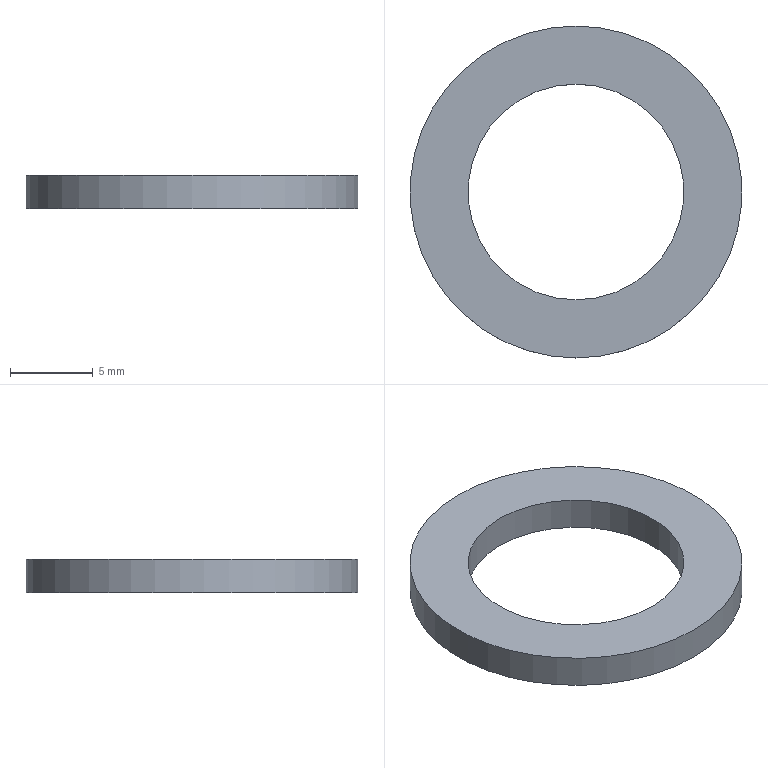Component | NX | GB-T848-2002_M12 | 1 solid | 4 faces | box 20 x 20 x 2 mm | volume 363 mm3 | cylinder 2 | plane 2 | commonest cylinder face diameters 20 x1 13 x1
STEP:
#1=CARTESIAN_POINT('',(0.,0.,0.));
#2=DIRECTION('',(0.,0.,1.));
#3=DIRECTION('',(1.,0.,0.));
#4=AXIS2_PLACEMENT_3D('',#1,#2,#3);
#5=CARTESIAN_POINT('',(0.,10.,-15.));
#6=VERTEX_POINT('',#5);
#7=CARTESIAN_POINT('',(0.,0.,-15.));
#8=DIRECTION('',(0.,0.,-1.));
#9=DIRECTION('',(0.,1.,0.));
#10=AXIS2_PLACEMENT_3D('',#7,#8,#9);
#11=CIRCLE('',#10,10.);
#12=CARTESIAN_POINT('',(0.,0.,-15.));
#13=DIRECTION('',(0.,0.,1.));
#14=DIRECTION('',(0.,-1.,0.));
#15=AXIS2_PLACEMENT_3D('',#12,#13,#14);
#16=CYLINDRICAL_SURFACE('',#15,10.);
#17=CARTESIAN_POINT('',(9.425,0.));
#18=DIRECTION('',(-1.,0.));
#19=VECTOR('',#18,1.);
#20=LINE('',#17,#19);
#21=(GEOMETRIC_REPRESENTATION_CONTEXT(2)PARAMETRIC_REPRESENTATION_CONTEXT()REPRESENTATION_CONTEXT('',''));
#22=DEFINITIONAL_REPRESENTATION('',(#20),#21);
#23=PCURVE('',#16,#22);
#24=CARTESIAN_POINT('',(0.,0.,-15.));
#25=DIRECTION('',(0.,0.,-1.));
#26=DIRECTION('',(0.,1.,0.));
#27=AXIS2_PLACEMENT_3D('',#24,#25,#26);
#28=PLANE('',#27);
#29=CARTESIAN_POINT('',(0.,0.));
#30=DIRECTION('',(1.,0.));
#31=AXIS2_PLACEMENT_2D('',#29,#30);
#32=CIRCLE('',#31,10.);
#33=(GEOMETRIC_REPRESENTATION_CONTEXT(2)PARAMETRIC_REPRESENTATION_CONTEXT()REPRESENTATION_CONTEXT('',''));
#34=DEFINITIONAL_REPRESENTATION('',(#32),#33);
#35=PCURVE('',#28,#34);
#36=SURFACE_CURVE('',#11,(#23,#35),.PCURVE_S1.);
#37=EDGE_CURVE('',#6,#6,#36,.T.);
#38=ORIENTED_EDGE('',*,*,#37,.F.);
#39=CARTESIAN_POINT('',(0.,10.,-13.));
#40=VERTEX_POINT('',#39);
#41=CARTESIAN_POINT('',(0.,10.,-15.));
#42=CARTESIAN_POINT('',(0.,10.,-13.));
#43=B_SPLINE_CURVE_WITH_KNOTS('',1,(#41,#42),.UNSPECIFIED.,.F.,.F.,(2,2),(0.,2.),.PIECEWISE_BEZIER_KNOTS.);
#44=CARTESIAN_POINT('',(9.425,0.));
#45=DIRECTION('',(0.,1.));
#46=VECTOR('',#45,1.);
#47=LINE('',#44,#46);
#48=(GEOMETRIC_REPRESENTATION_CONTEXT(2)PARAMETRIC_REPRESENTATION_CONTEXT()REPRESENTATION_CONTEXT('',''));
#49=DEFINITIONAL_REPRESENTATION('',(#47),#48);
#50=PCURVE('',#16,#49);
#51=CARTESIAN_POINT('',(3.142,0.));
#52=DIRECTION('',(0.,1.));
#53=VECTOR('',#52,1.);
#54=LINE('',#51,#53);
#55=(GEOMETRIC_REPRESENTATION_CONTEXT(2)PARAMETRIC_REPRESENTATION_CONTEXT()REPRESENTATION_CONTEXT('',''));
#56=DEFINITIONAL_REPRESENTATION('',(#54),#55);
#57=PCURVE('',#16,#56);
#58=SEAM_CURVE('',#43,(#50,#57),.PCURVE_S1.);
#59=EDGE_CURVE('',#6,#40,#58,.T.);
#60=ORIENTED_EDGE('',*,*,#59,.T.);
#61=CARTESIAN_POINT('',(0.,0.,-13.));
#62=DIRECTION('',(0.,0.,-1.));
#63=DIRECTION('',(0.,1.,0.));
#64=AXIS2_PLACEMENT_3D('',#61,#62,#63);
#65=CIRCLE('',#64,10.);
#66=CARTESIAN_POINT('',(9.425,2.));
#67=DIRECTION('',(-1.,0.));
#68=VECTOR('',#67,1.);
#69=LINE('',#66,#68);
#70=(GEOMETRIC_REPRESENTATION_CONTEXT(2)PARAMETRIC_REPRESENTATION_CONTEXT()REPRESENTATION_CONTEXT('',''));
#71=DEFINITIONAL_REPRESENTATION('',(#69),#70);
#72=PCURVE('',#16,#71);
#73=CARTESIAN_POINT('',(0.,0.,-13.));
#74=DIRECTION('',(0.,0.,-1.));
#75=DIRECTION('',(0.,1.,0.));
#76=AXIS2_PLACEMENT_3D('',#73,#74,#75);
#77=PLANE('',#76);
#78=CARTESIAN_POINT('',(0.,0.));
#79=DIRECTION('',(1.,0.));
#80=AXIS2_PLACEMENT_2D('',#78,#79);
#81=CIRCLE('',#80,10.);
#82=(GEOMETRIC_REPRESENTATION_CONTEXT(2)PARAMETRIC_REPRESENTATION_CONTEXT()REPRESENTATION_CONTEXT('',''));
#83=DEFINITIONAL_REPRESENTATION('',(#81),#82);
#84=PCURVE('',#77,#83);
#85=SURFACE_CURVE('',#65,(#72,#84),.PCURVE_S1.);
#86=EDGE_CURVE('',#40,#40,#85,.T.);
#87=ORIENTED_EDGE('',*,*,#86,.T.);
#88=ORIENTED_EDGE('',*,*,#59,.F.);
#89=EDGE_LOOP('',(#38,#60,#87,#88));
#90=FACE_BOUND('',#89,.T.);
#91=ADVANCED_FACE('',(#90),#16,.T.);
#92=CARTESIAN_POINT('',(0.,6.5,-15.));
#93=VERTEX_POINT('',#92);
#94=CARTESIAN_POINT('',(0.,0.,-15.));
#95=DIRECTION('',(0.,0.,-1.));
#96=DIRECTION('',(0.,1.,0.));
#97=AXIS2_PLACEMENT_3D('',#94,#95,#96);
#98=CIRCLE('',#97,6.5);
#99=CARTESIAN_POINT('',(0.,0.,-15.));
#100=DIRECTION('',(0.,0.,1.));
#101=DIRECTION('',(0.,-1.,0.));
#102=AXIS2_PLACEMENT_3D('',#99,#100,#101);
#103=CYLINDRICAL_SURFACE('',#102,6.5);
#104=CARTESIAN_POINT('',(9.425,0.));
#105=DIRECTION('',(-1.,0.));
#106=VECTOR('',#105,1.);
#107=LINE('',#104,#106);
#108=(GEOMETRIC_REPRESENTATION_CONTEXT(2)PARAMETRIC_REPRESENTATION_CONTEXT()REPRESENTATION_CONTEXT('',''));
#109=DEFINITIONAL_REPRESENTATION('',(#107),#108);
#110=PCURVE('',#103,#109);
#111=CARTESIAN_POINT('',(0.,0.));
#112=DIRECTION('',(1.,0.));
#113=AXIS2_PLACEMENT_2D('',#111,#112);
#114=CIRCLE('',#113,6.5);
#115=(GEOMETRIC_REPRESENTATION_CONTEXT(2)PARAMETRIC_REPRESENTATION_CONTEXT()REPRESENTATION_CONTEXT('',''));
#116=DEFINITIONAL_REPRESENTATION('',(#114),#115);
#117=PCURVE('',#28,#116);
#118=SURFACE_CURVE('',#98,(#110,#117),.PCURVE_S1.);
#119=EDGE_CURVE('',#93,#93,#118,.T.);
#120=ORIENTED_EDGE('',*,*,#119,.F.);
#121=CARTESIAN_POINT('',(0.,6.5,-13.));
#122=VERTEX_POINT('',#121);
#123=CARTESIAN_POINT('',(0.,6.5,-15.));
#124=CARTESIAN_POINT('',(0.,6.5,-13.));
#125=B_SPLINE_CURVE_WITH_KNOTS('',1,(#123,#124),.UNSPECIFIED.,.F.,.F.,(2,2),(0.,2.),.PIECEWISE_BEZIER_KNOTS.);
#126=CARTESIAN_POINT('',(9.425,0.));
#127=DIRECTION('',(0.,1.));
#128=VECTOR('',#127,1.);
#129=LINE('',#126,#128);
#130=(GEOMETRIC_REPRESENTATION_CONTEXT(2)PARAMETRIC_REPRESENTATION_CONTEXT()REPRESENTATION_CONTEXT('',''));
#131=DEFINITIONAL_REPRESENTATION('',(#129),#130);
#132=PCURVE('',#103,#131);
#133=CARTESIAN_POINT('',(3.142,0.));
#134=DIRECTION('',(0.,1.));
#135=VECTOR('',#134,1.);
#136=LINE('',#133,#135);
#137=(GEOMETRIC_REPRESENTATION_CONTEXT(2)PARAMETRIC_REPRESENTATION_CONTEXT()REPRESENTATION_CONTEXT('',''));
#138=DEFINITIONAL_REPRESENTATION('',(#136),#137);
#139=PCURVE('',#103,#138);
#140=SEAM_CURVE('',#125,(#132,#139),.PCURVE_S1.);
#141=EDGE_CURVE('',#93,#122,#140,.T.);
#142=ORIENTED_EDGE('',*,*,#141,.T.);
#143=CARTESIAN_POINT('',(0.,0.,-13.));
#144=DIRECTION('',(0.,0.,-1.));
#145=DIRECTION('',(0.,1.,0.));
#146=AXIS2_PLACEMENT_3D('',#143,#144,#145);
#147=CIRCLE('',#146,6.5);
#148=CARTESIAN_POINT('',(9.425,2.));
#149=DIRECTION('',(-1.,0.));
#150=VECTOR('',#149,1.);
#151=LINE('',#148,#150);
#152=(GEOMETRIC_REPRESENTATION_CONTEXT(2)PARAMETRIC_REPRESENTATION_CONTEXT()REPRESENTATION_CONTEXT('',''));
#153=DEFINITIONAL_REPRESENTATION('',(#151),#152);
#154=PCURVE('',#103,#153);
#155=CARTESIAN_POINT('',(0.,0.));
#156=DIRECTION('',(1.,0.));
#157=AXIS2_PLACEMENT_2D('',#155,#156);
#158=CIRCLE('',#157,6.5);
#159=(GEOMETRIC_REPRESENTATION_CONTEXT(2)PARAMETRIC_REPRESENTATION_CONTEXT()REPRESENTATION_CONTEXT('',''));
#160=DEFINITIONAL_REPRESENTATION('',(#158),#159);
#161=PCURVE('',#77,#160);
#162=SURFACE_CURVE('',#147,(#154,#161),.PCURVE_S1.);
#163=EDGE_CURVE('',#122,#122,#162,.T.);
#164=ORIENTED_EDGE('',*,*,#163,.T.);
#165=ORIENTED_EDGE('',*,*,#141,.F.);
#166=EDGE_LOOP('',(#120,#142,#164,#165));
#167=FACE_BOUND('',#166,.F.);
#168=ADVANCED_FACE('',(#167),#103,.F.);
#169=ORIENTED_EDGE('',*,*,#37,.T.);
#170=EDGE_LOOP('',(#169));
#171=FACE_BOUND('',#170,.T.);
#172=ORIENTED_EDGE('',*,*,#119,.F.);
#173=EDGE_LOOP('',(#172));
#174=FACE_BOUND('',#173,.T.);
#175=ADVANCED_FACE('',(#171,#174),#28,.T.);
#176=ORIENTED_EDGE('',*,*,#86,.F.);
#177=EDGE_LOOP('',(#176));
#178=FACE_BOUND('',#177,.T.);
#179=ORIENTED_EDGE('',*,*,#163,.T.);
#180=EDGE_LOOP('',(#179));
#181=FACE_BOUND('',#180,.T.);
#182=ADVANCED_FACE('',(#178,#181),#77,.F.);
#183=CLOSED_SHELL('',(#91,#168,#175,#182));
#184=MANIFOLD_SOLID_BREP('',#183);
#185=(LENGTH_UNIT()NAMED_UNIT(*)SI_UNIT(.MILLI.,.METRE.));
#186=UNCERTAINTY_MEASURE_WITH_UNIT(LENGTH_MEASURE(0.00001),#185,'','');
#187=(NAMED_UNIT(*)PLANE_ANGLE_UNIT()SI_UNIT($,.RADIAN.));
#188=(NAMED_UNIT(*)SI_UNIT($,.STERADIAN.)SOLID_ANGLE_UNIT());
#189=(GEOMETRIC_REPRESENTATION_CONTEXT(3)GLOBAL_UNCERTAINTY_ASSIGNED_CONTEXT((#186))GLOBAL_UNIT_ASSIGNED_CONTEXT((#185,#187,#188))REPRESENTATION_CONTEXT('',''));
#190=ADVANCED_BREP_SHAPE_REPRESENTATION('',(#4,#184),#189);